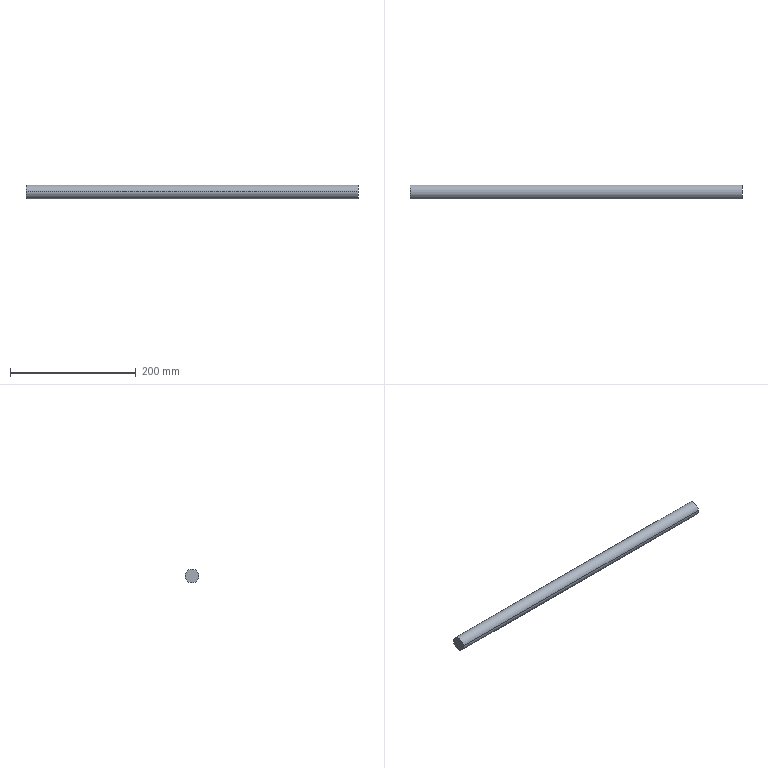Component | SolidWorks | DNR-71M20100BBEF2xx-A_504806-1_DNR-71M20100BBEF2xx-A_502906-1 | 1 solid | 4 faces | box 527.05 x 22.23 x 22.23 mm | volume 204468 mm3 | cylinder 2 | plane 2 | commonest cylinder face diameters 22.225 x2
build123d program:
from build123d import *

# Parameters (mm, degrees)
SKETCH1_R      = 11.113
EXTRUDE1_DEPTH = 263.525


with BuildPart() as part:
    # Sketch1 → Extrude1 (new, symmetric)
    with BuildSketch(Plane.XY):
        Circle(SKETCH1_R)
    extrude(amount=EXTRUDE1_DEPTH, both=True)


solid = part.part

# Placed as in the assembly
solid = solid.moved(Location((0, 49.445, 146.072), (0, 90, 0)))
STEP:
#1=COLOUR_RGB('',0.7922,0.8196,0.9333);
#2=FILL_AREA_STYLE_COLOUR('',#1);
#3=FILL_AREA_STYLE('',(#2));
#4=SURFACE_STYLE_FILL_AREA(#3);
#5=SURFACE_SIDE_STYLE('',(#4));
#6=SURFACE_STYLE_USAGE(.BOTH.,#5);
#7=PRESENTATION_STYLE_ASSIGNMENT((#6));
#8=CARTESIAN_POINT('',(10.375,1.512,5.803));
#9=VERTEX_POINT('',#8);
#10=CARTESIAN_POINT('',(10.375,2.381,5.699));
#11=VERTEX_POINT('',#10);
#12=CARTESIAN_POINT('',(10.375,1.947,5.751));
#13=DIRECTION('',(1.,0.,0.));
#14=DIRECTION('',(0.,-0.9928,0.1196));
#15=AXIS2_PLACEMENT_3D('',#12,#13,#14);
#16=CIRCLE('',#15,0.4375);
#17=EDGE_CURVE('',#9,#11,#16,.T.);
#18=ORIENTED_EDGE('',*,*,#17,.F.);
#19=CARTESIAN_POINT('',(-10.375,1.512,5.803));
#20=VERTEX_POINT('',#19);
#21=CARTESIAN_POINT('',(10.375,1.512,5.803));
#22=DIRECTION('',(-1.,-0.,-0.));
#23=VECTOR('',#22,39.37);
#24=LINE('',#21,#23);
#25=EDGE_CURVE('',#9,#20,#24,.T.);
#26=ORIENTED_EDGE('',*,*,#25,.T.);
#27=CARTESIAN_POINT('',(-10.375,2.381,5.699));
#28=VERTEX_POINT('',#27);
#29=CARTESIAN_POINT('',(-10.375,1.947,5.751));
#30=DIRECTION('',(1.,0.,0.));
#31=DIRECTION('',(0.,-0.9928,0.1196));
#32=AXIS2_PLACEMENT_3D('',#29,#30,#31);
#33=CIRCLE('',#32,0.4375);
#34=EDGE_CURVE('',#20,#28,#33,.T.);
#35=ORIENTED_EDGE('',*,*,#34,.T.);
#36=CARTESIAN_POINT('',(10.375,2.381,5.699));
#37=DIRECTION('',(-1.,-0.,-0.));
#38=VECTOR('',#37,39.37);
#39=LINE('',#36,#38);
#40=EDGE_CURVE('',#11,#28,#39,.T.);
#41=ORIENTED_EDGE('',*,*,#40,.F.);
#42=EDGE_LOOP('',(#18,#26,#35,#41));
#43=FACE_OUTER_BOUND('',#42,.T.);
#44=CARTESIAN_POINT('',(10.375,1.947,5.751));
#45=DIRECTION('',(-1.,-0.,-0.));
#46=DIRECTION('',(0.,0.9928,-0.1196));
#47=AXIS2_PLACEMENT_3D('',#44,#45,#46);
#48=CYLINDRICAL_SURFACE('',#47,0.4375);
#49=ADVANCED_FACE('',(#43),#48,.T.);
#50=ORIENTED_EDGE('',*,*,#25,.F.);
#51=CARTESIAN_POINT('',(10.375,1.947,5.751));
#52=DIRECTION('',(1.,0.,0.));
#53=DIRECTION('',(0.,-0.9928,0.1196));
#54=AXIS2_PLACEMENT_3D('',#51,#52,#53);
#55=CIRCLE('',#54,0.4375);
#56=EDGE_CURVE('',#11,#9,#55,.T.);
#57=ORIENTED_EDGE('',*,*,#56,.F.);
#58=ORIENTED_EDGE('',*,*,#40,.T.);
#59=CARTESIAN_POINT('',(-10.375,1.947,5.751));
#60=DIRECTION('',(1.,0.,0.));
#61=DIRECTION('',(0.,-0.9928,0.1196));
#62=AXIS2_PLACEMENT_3D('',#59,#60,#61);
#63=CIRCLE('',#62,0.4375);
#64=EDGE_CURVE('',#28,#20,#63,.T.);
#65=ORIENTED_EDGE('',*,*,#64,.T.);
#66=EDGE_LOOP('',(#50,#57,#58,#65));
#67=FACE_OUTER_BOUND('',#66,.T.);
#68=CARTESIAN_POINT('',(10.375,1.947,5.751));
#69=DIRECTION('',(-1.,-0.,-0.));
#70=DIRECTION('',(0.,0.9928,-0.1196));
#71=AXIS2_PLACEMENT_3D('',#68,#69,#70);
#72=CYLINDRICAL_SURFACE('',#71,0.4375);
#73=ADVANCED_FACE('',(#67),#72,.T.);
#74=ORIENTED_EDGE('',*,*,#56,.T.);
#75=ORIENTED_EDGE('',*,*,#17,.T.);
#76=EDGE_LOOP('',(#74,#75));
#77=FACE_OUTER_BOUND('',#76,.T.);
#78=CARTESIAN_POINT('',(10.375,1.947,5.751));
#79=DIRECTION('',(1.,0.,0.));
#80=DIRECTION('',(-0.,-0.9928,0.1196));
#81=AXIS2_PLACEMENT_3D('',#78,#79,#80);
#82=PLANE('',#81);
#83=ADVANCED_FACE('',(#77),#82,.T.);
#84=ORIENTED_EDGE('',*,*,#64,.F.);
#85=ORIENTED_EDGE('',*,*,#34,.F.);
#86=EDGE_LOOP('',(#84,#85));
#87=FACE_OUTER_BOUND('',#86,.T.);
#88=CARTESIAN_POINT('',(-10.375,1.947,5.751));
#89=DIRECTION('',(1.,0.,0.));
#90=DIRECTION('',(-0.,-0.9928,0.1196));
#91=AXIS2_PLACEMENT_3D('',#88,#89,#90);
#92=PLANE('',#91);
#93=ADVANCED_FACE('',(#87),#92,.F.);
#94=CLOSED_SHELL('',(#49,#73,#83,#93));
#95=MANIFOLD_SOLID_BREP('',#94);
#96=STYLED_ITEM('',(#7),#95);
#97=PRESENTATION_LAYER_ASSIGNMENT('','',(#96));
#98=CARTESIAN_POINT('',(0.,0.,0.));
#99=DIRECTION('',(0.,0.,1.));
#100=DIRECTION('',(1.,0.,0.));
#101=AXIS2_PLACEMENT_3D('',#98,#99,#100);
#102=(LENGTH_UNIT()NAMED_UNIT(*)SI_UNIT($,.METRE.));
#103=LENGTH_MEASURE_WITH_UNIT(LENGTH_MEASURE(0.0254),#102);
#104=DIMENSIONAL_EXPONENTS(1.,0.,0.,0.,0.,0.,0.);
#105=(CONVERSION_BASED_UNIT('',#103)LENGTH_UNIT()NAMED_UNIT(#104));
#106=UNCERTAINTY_MEASURE_WITH_UNIT(LENGTH_MEASURE(0.00001),#105,'','');
#107=(NAMED_UNIT(*)PLANE_ANGLE_UNIT()SI_UNIT($,.RADIAN.));
#108=(NAMED_UNIT(*)SI_UNIT($,.STERADIAN.)SOLID_ANGLE_UNIT());
#109=(GEOMETRIC_REPRESENTATION_CONTEXT(3)GLOBAL_UNCERTAINTY_ASSIGNED_CONTEXT((#106))GLOBAL_UNIT_ASSIGNED_CONTEXT((#105,#107,#108))REPRESENTATION_CONTEXT('',''));
#110=ADVANCED_BREP_SHAPE_REPRESENTATION('',(#95,#101),#109);
#111=(LENGTH_UNIT()NAMED_UNIT(*)SI_UNIT($,.METRE.));
#112=LENGTH_MEASURE_WITH_UNIT(LENGTH_MEASURE(0.0254),#111);
#113=DIMENSIONAL_EXPONENTS(1.,0.,0.,0.,0.,0.,0.);
#114=(CONVERSION_BASED_UNIT('',#112)LENGTH_UNIT()NAMED_UNIT(#113));
#115=UNCERTAINTY_MEASURE_WITH_UNIT(LENGTH_MEASURE(0.00001),#114,'','');
#116=(NAMED_UNIT(*)PLANE_ANGLE_UNIT()SI_UNIT($,.RADIAN.));
#117=(NAMED_UNIT(*)SI_UNIT($,.STERADIAN.)SOLID_ANGLE_UNIT());
#118=(GEOMETRIC_REPRESENTATION_CONTEXT(3)GLOBAL_UNCERTAINTY_ASSIGNED_CONTEXT((#115))GLOBAL_UNIT_ASSIGNED_CONTEXT((#114,#116,#117))REPRESENTATION_CONTEXT('',''));
#119=MECHANICAL_DESIGN_GEOMETRIC_PRESENTATION_REPRESENTATION('',(#96),#118);